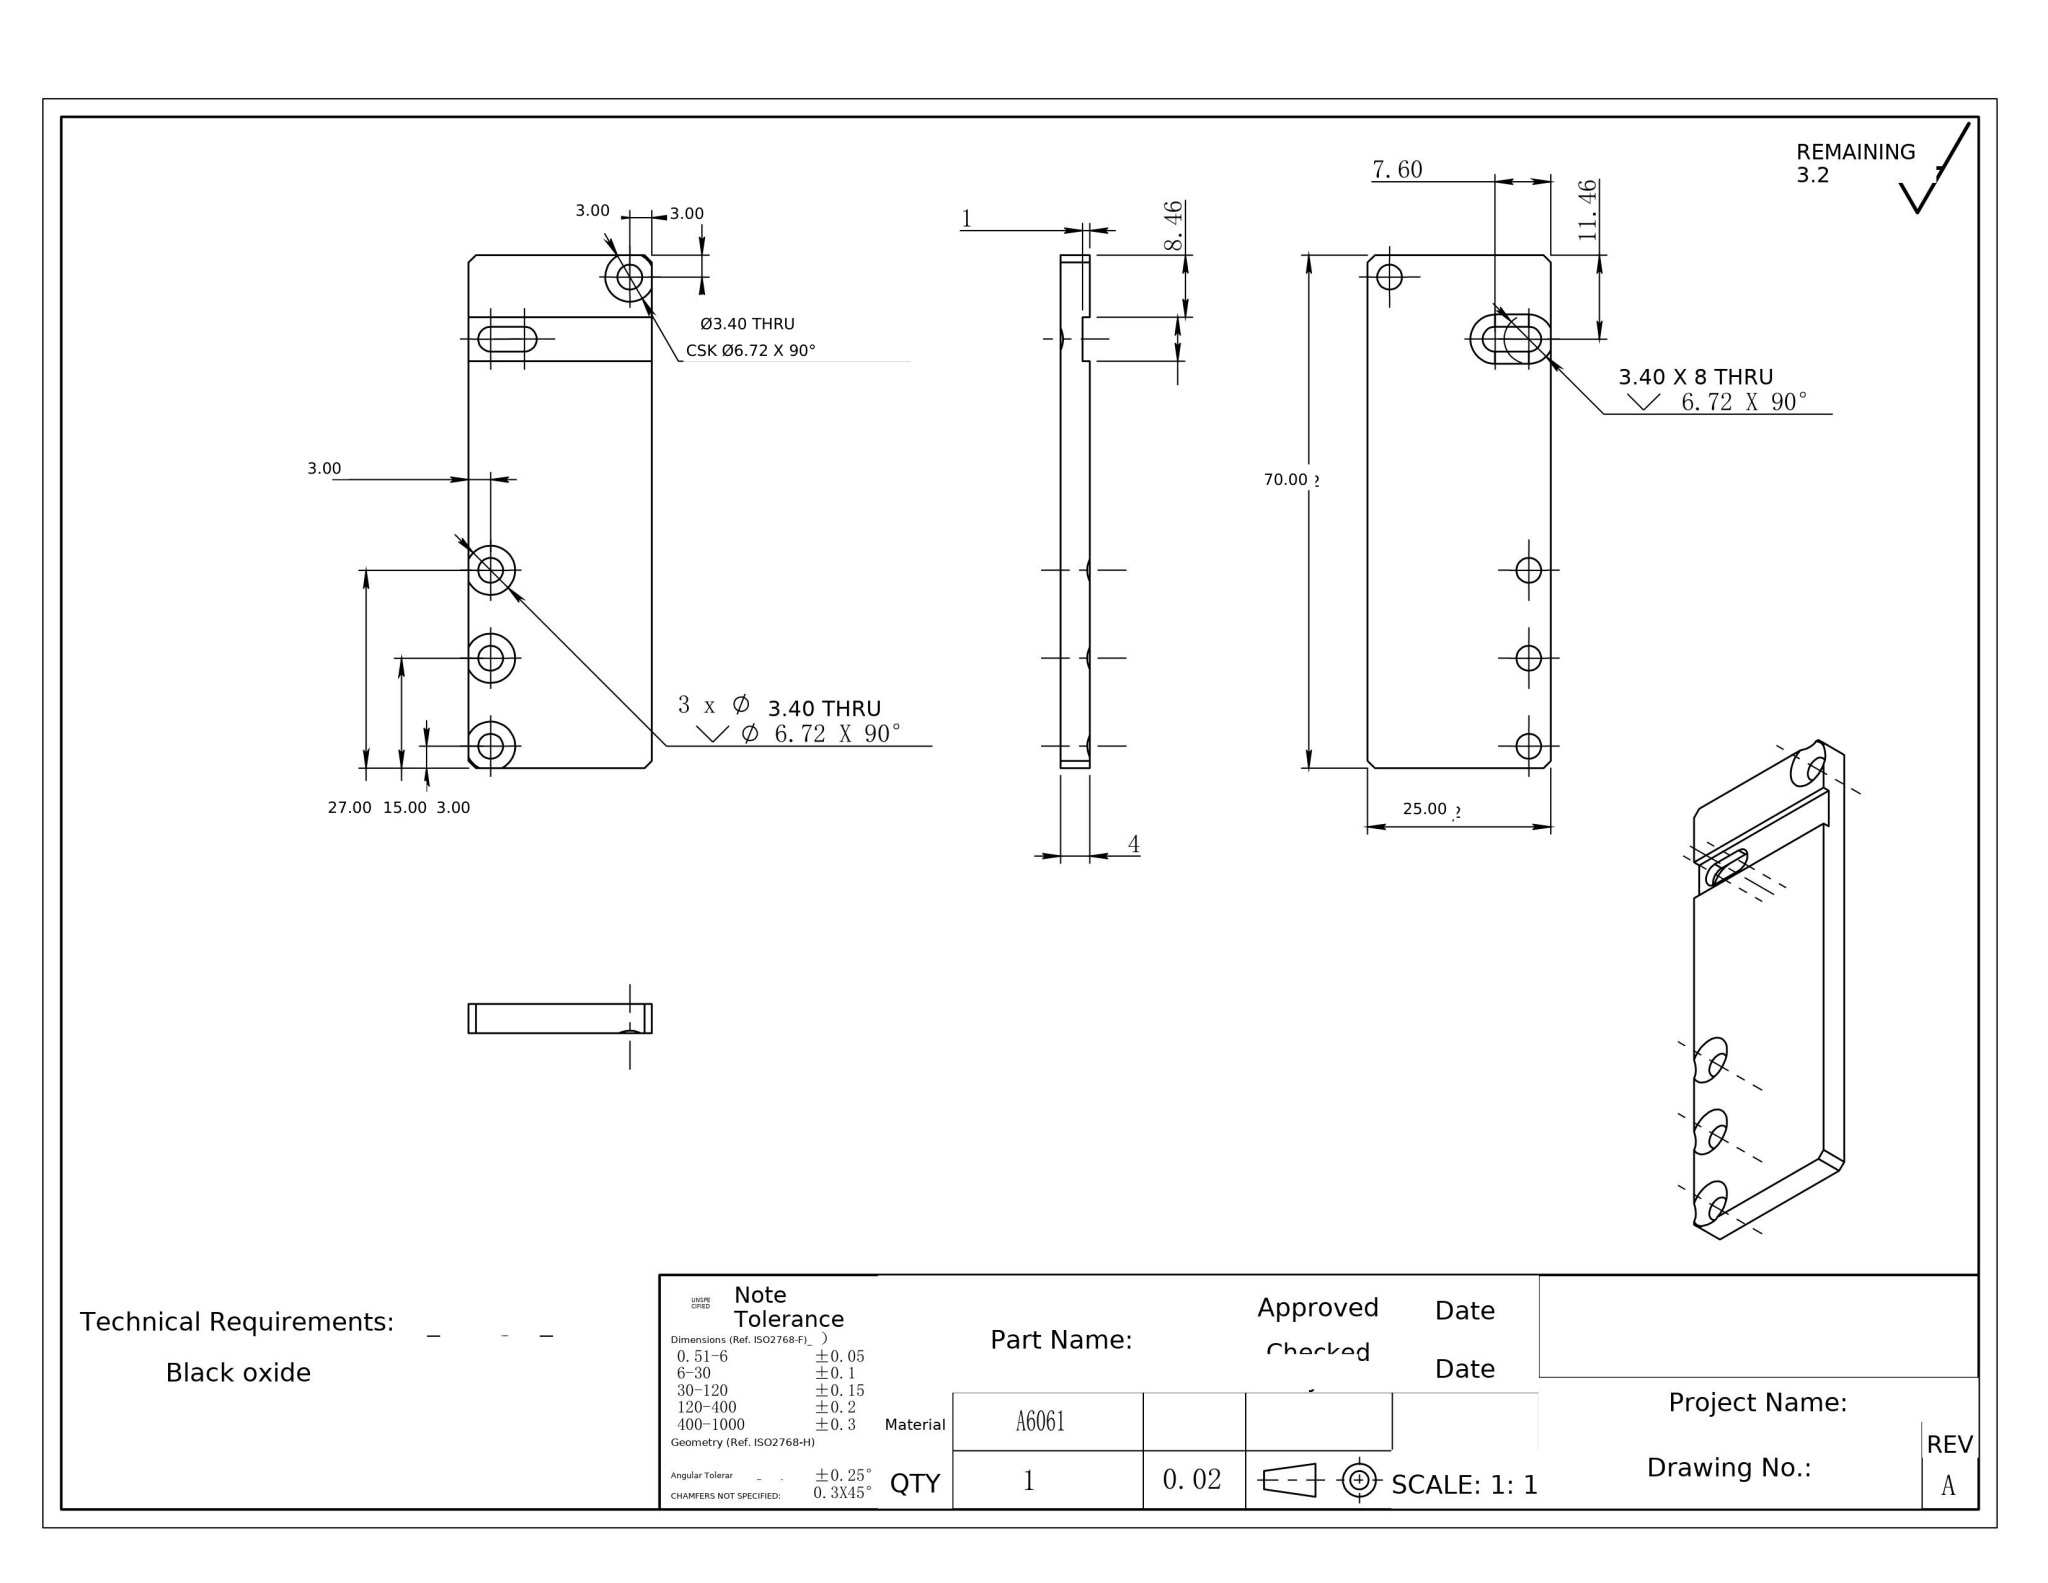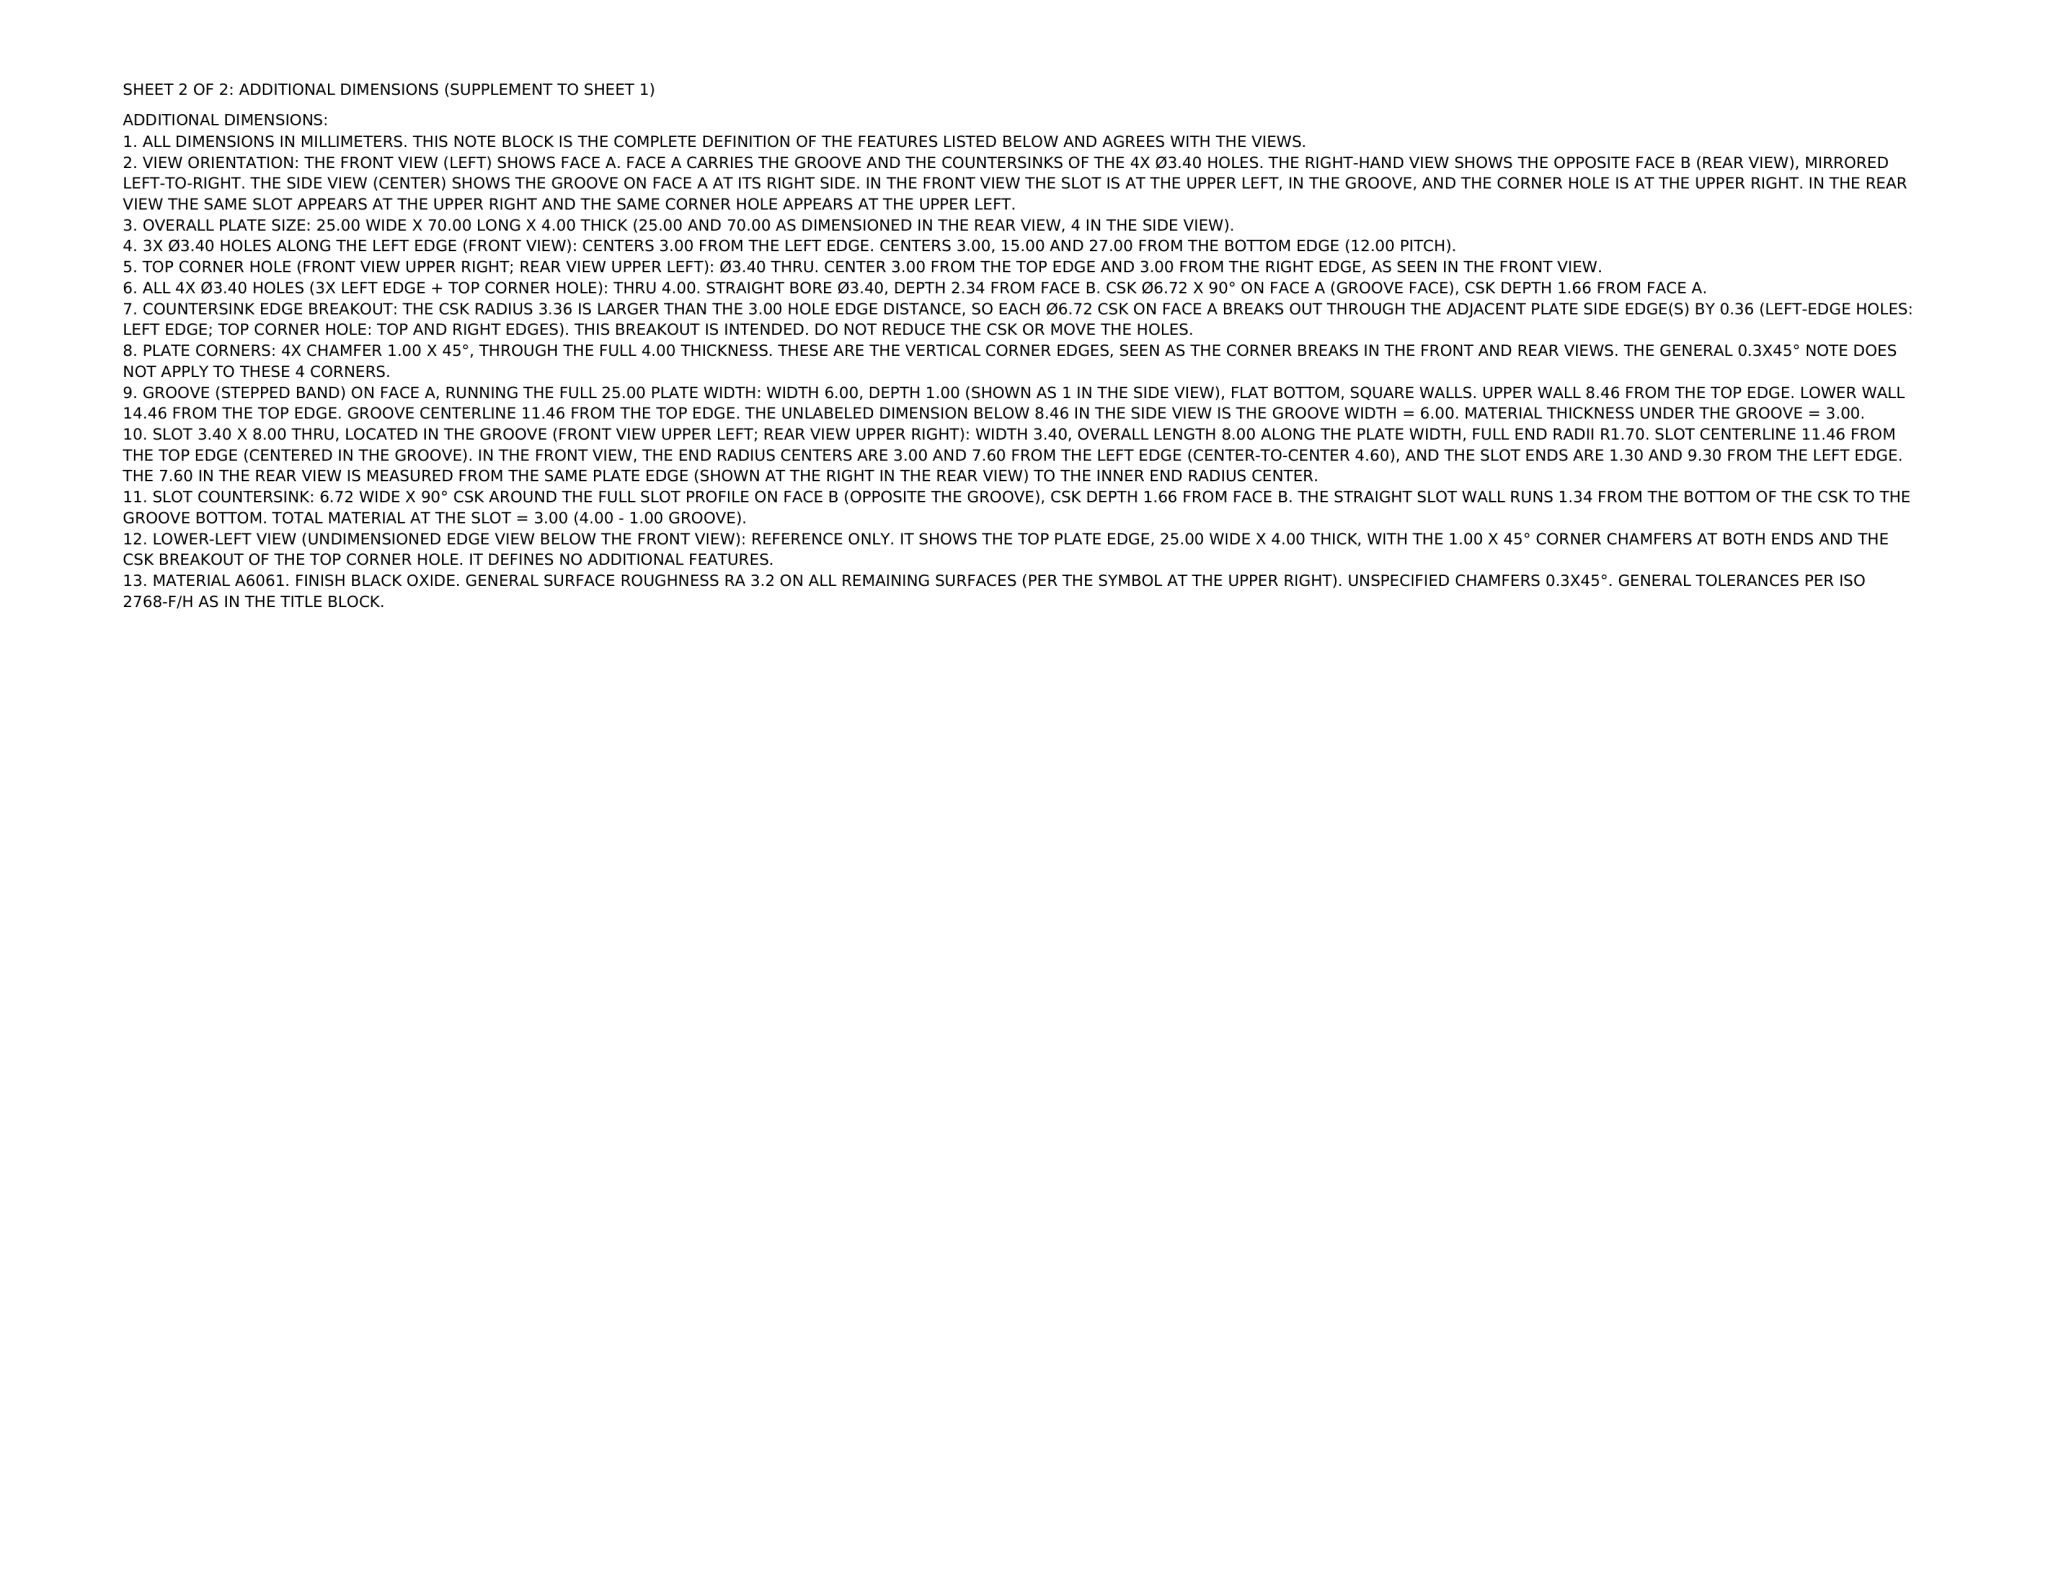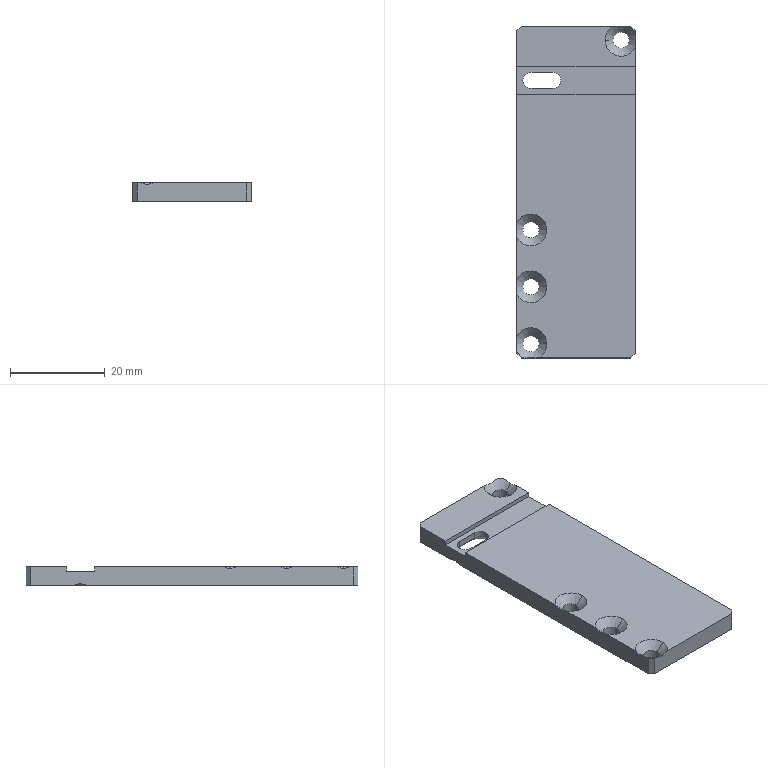Part | NX | mm | 1 solid | 42 faces | box 25 x 70 x 4 mm | volume 6513 mm3 | plane 20 | cylinder 11 | cone 11 | commonest cylinder face diameters 3.4 x11